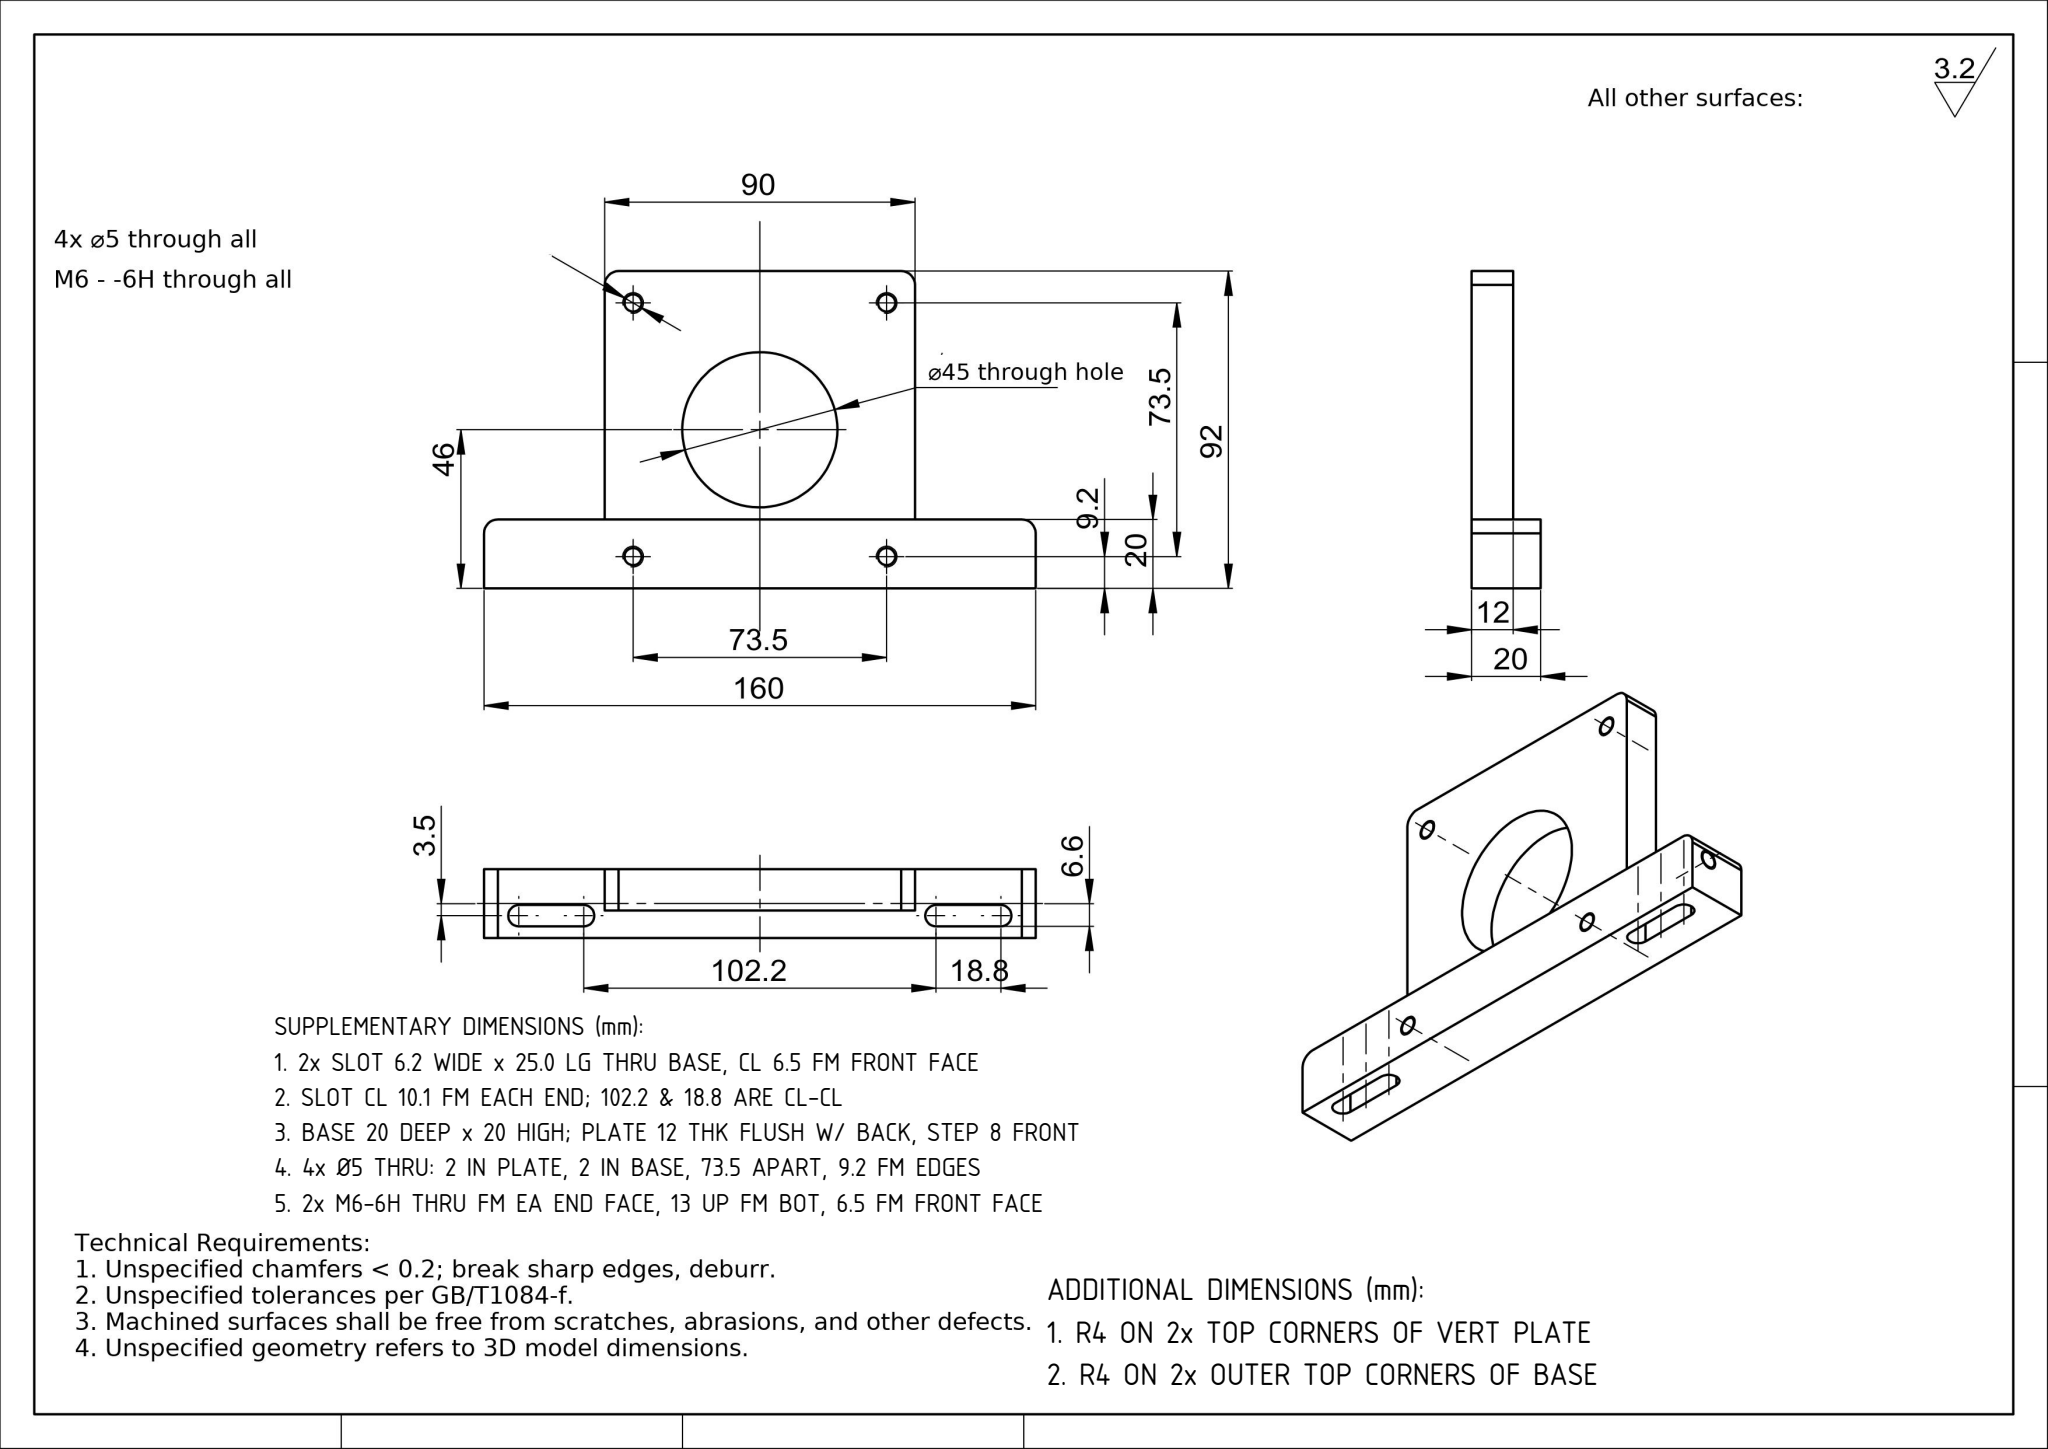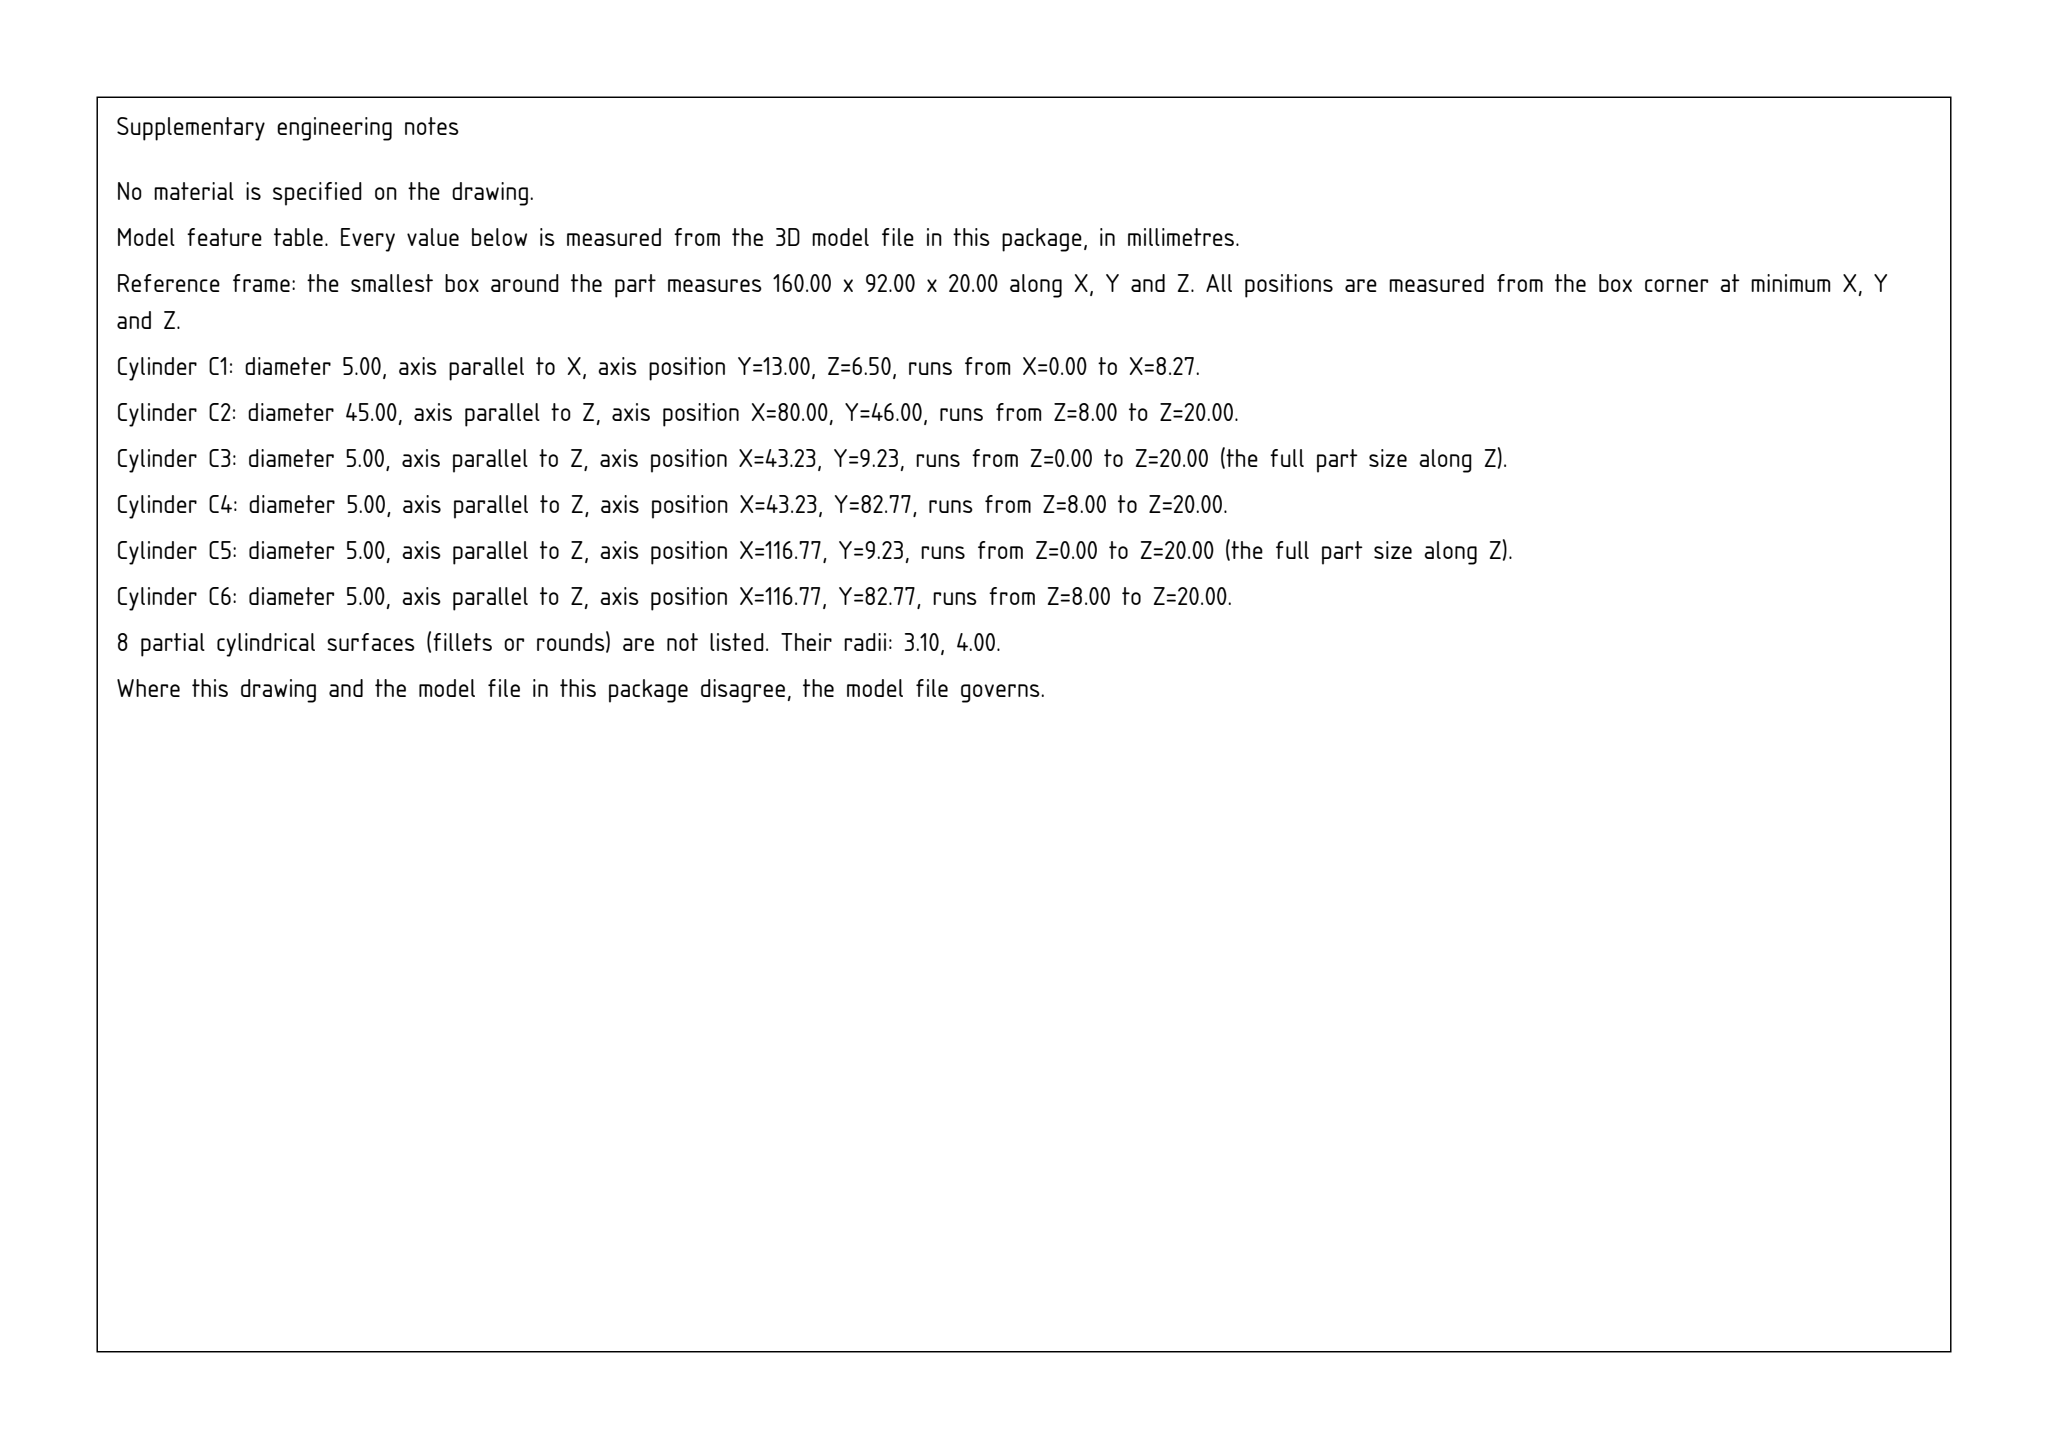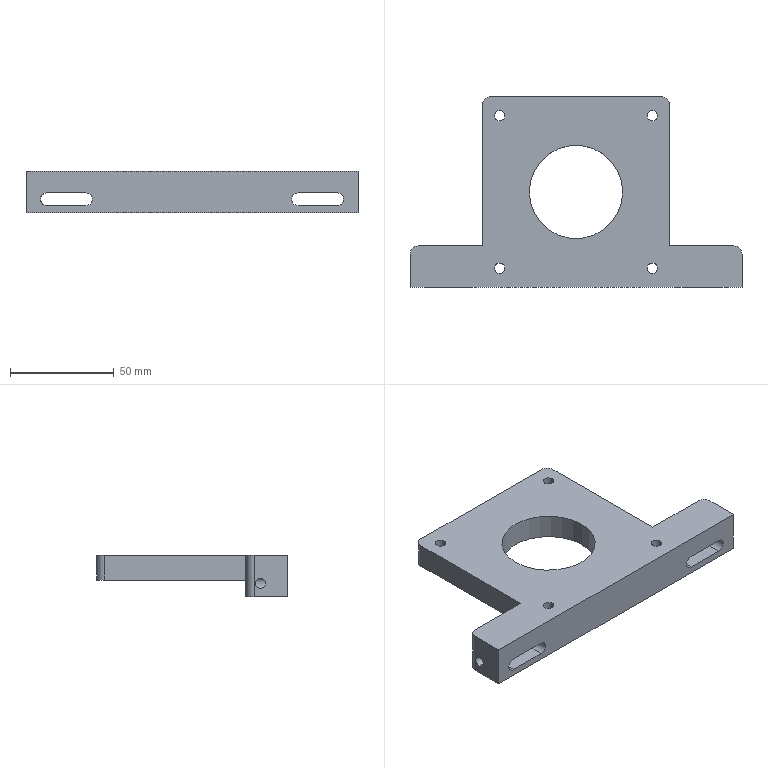Part | SolidWorks | mm | 1 solid | 34 faces | box 160 x 92 x 20 mm | volume 115186 mm3 | cylinder 20 | plane 14 | commonest cylinder face diameters 5 x10 6.2 x4 8 x4 45 x2